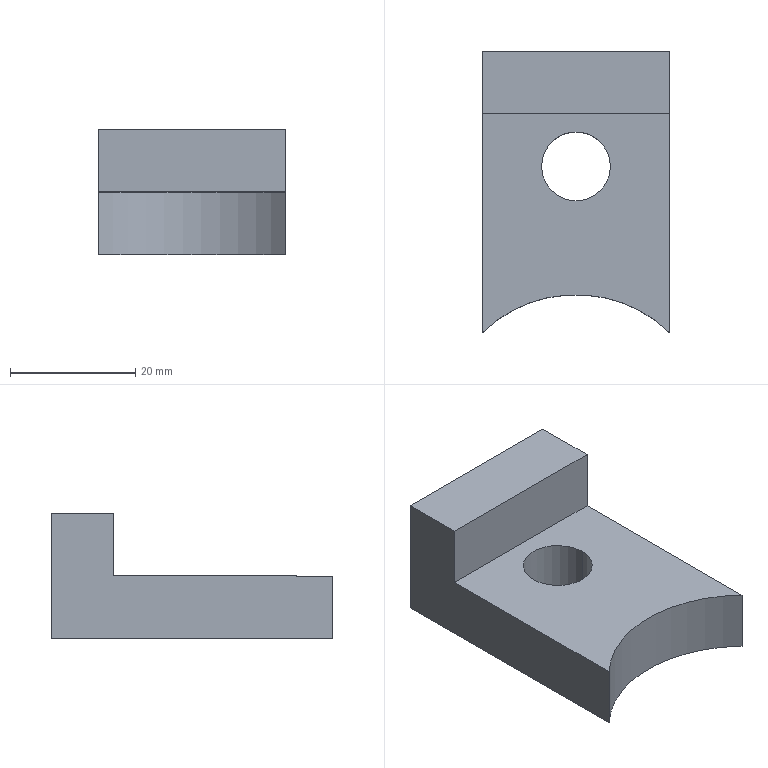Component | SolidWorks | DoubleFilmTransport-1_FlangeClamp-1 | 1 solid | 10 faces | box 30 x 45 x 20 mm | volume 14291 mm3 | plane 7 | cylinder 3 | commonest cylinder face diameters 11 x2 43 x1
build123d program:
from build123d import *

# Parameters (mm, degrees)
BOSS_EXTRUDE1_DEPTH            = 10
SKETCH2_W                      = 30
SKETCH2_H                      = 10
BOSS_EXTRUDE2_DEPTH            = 10
F_11_0_11_DIAMETER_HOLE1_D     = 11
F_11_0_11_DIAMETER_HOLE1_DEPTH = 20


with BuildPart() as part:
    # Sketch1 → Boss-Extrude1 (new body)
    with BuildSketch(Plane(origin=(10, 0, 0), x_dir=(0, 0, -1), z_dir=(1, 0, 0))):
        with BuildLine():
            Line((-15, 0), (-15, -45))
            ThreePointArc((-15, -45), (0, -38.903), (15, -45))
            Line((15, -45), (15, 0))
            Line((15, 0), (-15, 0))
        make_face()
    extrude(amount=-BOSS_EXTRUDE1_DEPTH)

    # Sketch2 → Boss-Extrude2 (add)
    with BuildSketch(Plane(origin=(10, 0, 0), x_dir=(0, 0, -1), z_dir=(1, 0, 0))):
        with Locations((0, -5)):
            Rectangle(SKETCH2_W, SKETCH2_H)
    extrude(amount=BOSS_EXTRUDE2_DEPTH)

    # 11.0 _11_ Diameter Hole1
    with Locations(Plane.ZY):
        with Locations((0, -18.403)):
            Hole(F_11_0_11_DIAMETER_HOLE1_D / 2, depth=F_11_0_11_DIAMETER_HOLE1_DEPTH)


solid = part.part

# Placed as in the assembly
solid = solid.moved(Location((-384.677, 143.776, 56), (0, -90, 0)))
STEP:
#1=COLOUR_RGB('',0.7922,0.8196,0.9333);
#2=FILL_AREA_STYLE_COLOUR('',#1);
#3=FILL_AREA_STYLE('',(#2));
#4=SURFACE_STYLE_FILL_AREA(#3);
#5=SURFACE_SIDE_STYLE('',(#4));
#6=SURFACE_STYLE_USAGE(.BOTH.,#5);
#7=PRESENTATION_STYLE_ASSIGNMENT((#6));
#8=CARTESIAN_POINT('',(-14.928,4.936,2.598));
#9=VERTEX_POINT('',#8);
#10=CARTESIAN_POINT('',(-15.361,4.936,2.598));
#11=VERTEX_POINT('',#10);
#12=CARTESIAN_POINT('',(-15.145,4.936,2.598));
#13=DIRECTION('',(-0.,0.,-1.));
#14=DIRECTION('',(-1.,0.,0.));
#15=AXIS2_PLACEMENT_3D('',#12,#13,#14);
#16=CIRCLE('',#15,0.2165);
#17=EDGE_CURVE('',#9,#11,#16,.T.);
#18=ORIENTED_EDGE('',*,*,#17,.F.);
#19=CARTESIAN_POINT('',(-14.928,4.936,2.205));
#20=VERTEX_POINT('',#19);
#21=CARTESIAN_POINT('',(-14.928,4.936,2.205));
#22=DIRECTION('',(-0.,0.,-1.));
#23=VECTOR('',#22,39.37);
#24=LINE('',#21,#23);
#25=EDGE_CURVE('',#9,#20,#24,.T.);
#26=ORIENTED_EDGE('',*,*,#25,.T.);
#27=CARTESIAN_POINT('',(-15.361,4.936,2.205));
#28=VERTEX_POINT('',#27);
#29=CARTESIAN_POINT('',(-15.145,4.936,2.205));
#30=DIRECTION('',(-0.,0.,-1.));
#31=DIRECTION('',(-1.,0.,0.));
#32=AXIS2_PLACEMENT_3D('',#29,#30,#31);
#33=CIRCLE('',#32,0.2165);
#34=EDGE_CURVE('',#20,#28,#33,.T.);
#35=ORIENTED_EDGE('',*,*,#34,.T.);
#36=CARTESIAN_POINT('',(-15.361,4.936,2.205));
#37=DIRECTION('',(-0.,0.,-1.));
#38=VECTOR('',#37,39.37);
#39=LINE('',#36,#38);
#40=EDGE_CURVE('',#11,#28,#39,.T.);
#41=ORIENTED_EDGE('',*,*,#40,.F.);
#42=EDGE_LOOP('',(#18,#26,#35,#41));
#43=FACE_OUTER_BOUND('',#42,.T.);
#44=CARTESIAN_POINT('',(-15.145,4.936,2.205));
#45=DIRECTION('',(-0.,0.,-1.));
#46=DIRECTION('',(-1.,0.,0.));
#47=AXIS2_PLACEMENT_3D('',#44,#45,#46);
#48=CYLINDRICAL_SURFACE('',#47,0.2165);
#49=ADVANCED_FACE('',(#43),#48,.F.);
#50=CARTESIAN_POINT('',(-15.145,4.936,2.598));
#51=DIRECTION('',(-0.,0.,-1.));
#52=DIRECTION('',(-1.,0.,0.));
#53=AXIS2_PLACEMENT_3D('',#50,#51,#52);
#54=CIRCLE('',#53,0.2165);
#55=EDGE_CURVE('',#11,#9,#54,.T.);
#56=ORIENTED_EDGE('',*,*,#55,.T.);
#57=ORIENTED_EDGE('',*,*,#17,.T.);
#58=EDGE_LOOP('',(#56,#57));
#59=FACE_BOUND('',#58,.T.);
#60=CARTESIAN_POINT('',(-15.735,5.267,2.598));
#61=VERTEX_POINT('',#60);
#62=CARTESIAN_POINT('',(-14.554,5.267,2.598));
#63=VERTEX_POINT('',#62);
#64=CARTESIAN_POINT('',(-14.554,5.267,2.598));
#65=DIRECTION('',(1.,0.,0.));
#66=VECTOR('',#65,39.37);
#67=LINE('',#64,#66);
#68=EDGE_CURVE('',#61,#63,#67,.T.);
#69=ORIENTED_EDGE('',*,*,#68,.F.);
#70=CARTESIAN_POINT('',(-15.735,3.889,2.598));
#71=VERTEX_POINT('',#70);
#72=CARTESIAN_POINT('',(-15.735,5.66,2.598));
#73=DIRECTION('',(0.,-1.,-0.));
#74=VECTOR('',#73,39.37);
#75=LINE('',#72,#74);
#76=EDGE_CURVE('',#61,#71,#75,.T.);
#77=ORIENTED_EDGE('',*,*,#76,.T.);
#78=CARTESIAN_POINT('',(-14.554,3.889,2.598));
#79=VERTEX_POINT('',#78);
#80=CARTESIAN_POINT('',(-15.145,3.282,2.598));
#81=DIRECTION('',(-0.,0.,-1.));
#82=DIRECTION('',(-1.,0.,0.));
#83=AXIS2_PLACEMENT_3D('',#80,#81,#82);
#84=CIRCLE('',#83,0.8465);
#85=EDGE_CURVE('',#71,#79,#84,.T.);
#86=ORIENTED_EDGE('',*,*,#85,.T.);
#87=CARTESIAN_POINT('',(-14.554,3.889,2.598));
#88=DIRECTION('',(-0.,1.,0.));
#89=VECTOR('',#88,39.37);
#90=LINE('',#87,#89);
#91=EDGE_CURVE('',#79,#63,#90,.T.);
#92=ORIENTED_EDGE('',*,*,#91,.T.);
#93=EDGE_LOOP('',(#69,#77,#86,#92));
#94=FACE_OUTER_BOUND('',#93,.T.);
#95=CARTESIAN_POINT('',(-15.145,3.282,2.598));
#96=DIRECTION('',(-0.,0.,-1.));
#97=DIRECTION('',(-1.,-0.,0.));
#98=AXIS2_PLACEMENT_3D('',#95,#96,#97);
#99=PLANE('',#98);
#100=ADVANCED_FACE('',(#59,#94),#99,.F.);
#101=CARTESIAN_POINT('',(-15.735,5.66,2.205));
#102=VERTEX_POINT('',#101);
#103=CARTESIAN_POINT('',(-15.735,5.66,2.992));
#104=VERTEX_POINT('',#103);
#105=CARTESIAN_POINT('',(-15.735,5.66,2.205));
#106=DIRECTION('',(0.,-0.,1.));
#107=VECTOR('',#106,39.37);
#108=LINE('',#105,#107);
#109=EDGE_CURVE('',#102,#104,#108,.T.);
#110=ORIENTED_EDGE('',*,*,#109,.T.);
#111=CARTESIAN_POINT('',(-14.554,5.66,2.992));
#112=VERTEX_POINT('',#111);
#113=CARTESIAN_POINT('',(-15.735,5.66,2.992));
#114=DIRECTION('',(-1.,-0.,0.));
#115=VECTOR('',#114,39.37);
#116=LINE('',#113,#115);
#117=EDGE_CURVE('',#112,#104,#116,.T.);
#118=ORIENTED_EDGE('',*,*,#117,.F.);
#119=CARTESIAN_POINT('',(-14.554,5.66,2.205));
#120=VERTEX_POINT('',#119);
#121=CARTESIAN_POINT('',(-14.554,5.66,2.205));
#122=DIRECTION('',(0.,-0.,1.));
#123=VECTOR('',#122,39.37);
#124=LINE('',#121,#123);
#125=EDGE_CURVE('',#120,#112,#124,.T.);
#126=ORIENTED_EDGE('',*,*,#125,.F.);
#127=CARTESIAN_POINT('',(-14.554,5.66,2.205));
#128=DIRECTION('',(-1.,-0.,0.));
#129=VECTOR('',#128,39.37);
#130=LINE('',#127,#129);
#131=EDGE_CURVE('',#120,#102,#130,.T.);
#132=ORIENTED_EDGE('',*,*,#131,.T.);
#133=EDGE_LOOP('',(#110,#118,#126,#132));
#134=FACE_OUTER_BOUND('',#133,.T.);
#135=CARTESIAN_POINT('',(-14.554,5.66,2.205));
#136=DIRECTION('',(-0.,1.,0.));
#137=DIRECTION('',(-1.,-0.,0.));
#138=AXIS2_PLACEMENT_3D('',#135,#136,#137);
#139=PLANE('',#138);
#140=ADVANCED_FACE('',(#134),#139,.T.);
#141=ORIENTED_EDGE('',*,*,#91,.F.);
#142=CARTESIAN_POINT('',(-14.554,3.889,2.205));
#143=VERTEX_POINT('',#142);
#144=CARTESIAN_POINT('',(-14.554,3.889,2.205));
#145=DIRECTION('',(0.,-0.,1.));
#146=VECTOR('',#145,39.37);
#147=LINE('',#144,#146);
#148=EDGE_CURVE('',#143,#79,#147,.T.);
#149=ORIENTED_EDGE('',*,*,#148,.F.);
#150=CARTESIAN_POINT('',(-14.554,3.889,2.205));
#151=DIRECTION('',(-0.,1.,0.));
#152=VECTOR('',#151,39.37);
#153=LINE('',#150,#152);
#154=EDGE_CURVE('',#143,#120,#153,.T.);
#155=ORIENTED_EDGE('',*,*,#154,.T.);
#156=ORIENTED_EDGE('',*,*,#125,.T.);
#157=CARTESIAN_POINT('',(-14.554,5.267,2.992));
#158=VERTEX_POINT('',#157);
#159=CARTESIAN_POINT('',(-14.554,5.66,2.992));
#160=DIRECTION('',(-0.,1.,0.));
#161=VECTOR('',#160,39.37);
#162=LINE('',#159,#161);
#163=EDGE_CURVE('',#158,#112,#162,.T.);
#164=ORIENTED_EDGE('',*,*,#163,.F.);
#165=CARTESIAN_POINT('',(-14.554,5.267,2.992));
#166=DIRECTION('',(-0.,0.,-1.));
#167=VECTOR('',#166,39.37);
#168=LINE('',#165,#167);
#169=EDGE_CURVE('',#158,#63,#168,.T.);
#170=ORIENTED_EDGE('',*,*,#169,.T.);
#171=EDGE_LOOP('',(#141,#149,#155,#156,#164,#170));
#172=FACE_OUTER_BOUND('',#171,.T.);
#173=CARTESIAN_POINT('',(-14.554,3.889,2.205));
#174=DIRECTION('',(1.,0.,-0.));
#175=DIRECTION('',(-0.,0.,-1.));
#176=AXIS2_PLACEMENT_3D('',#173,#174,#175);
#177=PLANE('',#176);
#178=ADVANCED_FACE('',(#172),#177,.T.);
#179=ORIENTED_EDGE('',*,*,#85,.F.);
#180=CARTESIAN_POINT('',(-15.735,3.889,2.205));
#181=VERTEX_POINT('',#180);
#182=CARTESIAN_POINT('',(-15.735,3.889,2.205));
#183=DIRECTION('',(0.,-0.,1.));
#184=VECTOR('',#183,39.37);
#185=LINE('',#182,#184);
#186=EDGE_CURVE('',#181,#71,#185,.T.);
#187=ORIENTED_EDGE('',*,*,#186,.F.);
#188=CARTESIAN_POINT('',(-15.145,3.282,2.205));
#189=DIRECTION('',(-0.,0.,-1.));
#190=DIRECTION('',(-1.,0.,0.));
#191=AXIS2_PLACEMENT_3D('',#188,#189,#190);
#192=CIRCLE('',#191,0.8465);
#193=EDGE_CURVE('',#181,#143,#192,.T.);
#194=ORIENTED_EDGE('',*,*,#193,.T.);
#195=ORIENTED_EDGE('',*,*,#148,.T.);
#196=EDGE_LOOP('',(#179,#187,#194,#195));
#197=FACE_OUTER_BOUND('',#196,.T.);
#198=CARTESIAN_POINT('',(-15.145,3.282,2.205));
#199=DIRECTION('',(0.,-0.,1.));
#200=DIRECTION('',(1.,0.,0.));
#201=AXIS2_PLACEMENT_3D('',#198,#199,#200);
#202=CYLINDRICAL_SURFACE('',#201,0.8465);
#203=ADVANCED_FACE('',(#197),#202,.F.);
#204=ORIENTED_EDGE('',*,*,#76,.F.);
#205=CARTESIAN_POINT('',(-15.735,5.267,2.992));
#206=VERTEX_POINT('',#205);
#207=CARTESIAN_POINT('',(-15.735,5.267,2.992));
#208=DIRECTION('',(-0.,0.,-1.));
#209=VECTOR('',#208,39.37);
#210=LINE('',#207,#209);
#211=EDGE_CURVE('',#206,#61,#210,.T.);
#212=ORIENTED_EDGE('',*,*,#211,.F.);
#213=CARTESIAN_POINT('',(-15.735,5.267,2.992));
#214=DIRECTION('',(0.,-1.,-0.));
#215=VECTOR('',#214,39.37);
#216=LINE('',#213,#215);
#217=EDGE_CURVE('',#104,#206,#216,.T.);
#218=ORIENTED_EDGE('',*,*,#217,.F.);
#219=ORIENTED_EDGE('',*,*,#109,.F.);
#220=CARTESIAN_POINT('',(-15.735,5.66,2.205));
#221=DIRECTION('',(0.,-1.,-0.));
#222=VECTOR('',#221,39.37);
#223=LINE('',#220,#222);
#224=EDGE_CURVE('',#102,#181,#223,.T.);
#225=ORIENTED_EDGE('',*,*,#224,.T.);
#226=ORIENTED_EDGE('',*,*,#186,.T.);
#227=EDGE_LOOP('',(#204,#212,#218,#219,#225,#226));
#228=FACE_OUTER_BOUND('',#227,.T.);
#229=CARTESIAN_POINT('',(-15.735,5.66,2.205));
#230=DIRECTION('',(-1.,-0.,-0.));
#231=DIRECTION('',(0.,-1.,-0.));
#232=AXIS2_PLACEMENT_3D('',#229,#230,#231);
#233=PLANE('',#232);
#234=ADVANCED_FACE('',(#228),#233,.T.);
#235=CARTESIAN_POINT('',(-15.145,4.936,2.205));
#236=DIRECTION('',(-0.,0.,-1.));
#237=DIRECTION('',(-1.,0.,0.));
#238=AXIS2_PLACEMENT_3D('',#235,#236,#237);
#239=CIRCLE('',#238,0.2165);
#240=EDGE_CURVE('',#28,#20,#239,.T.);
#241=ORIENTED_EDGE('',*,*,#240,.F.);
#242=ORIENTED_EDGE('',*,*,#34,.F.);
#243=EDGE_LOOP('',(#241,#242));
#244=FACE_BOUND('',#243,.T.);
#245=ORIENTED_EDGE('',*,*,#131,.F.);
#246=ORIENTED_EDGE('',*,*,#154,.F.);
#247=ORIENTED_EDGE('',*,*,#193,.F.);
#248=ORIENTED_EDGE('',*,*,#224,.F.);
#249=EDGE_LOOP('',(#245,#246,#247,#248));
#250=FACE_OUTER_BOUND('',#249,.T.);
#251=CARTESIAN_POINT('',(-15.145,3.282,2.205));
#252=DIRECTION('',(-0.,0.,-1.));
#253=DIRECTION('',(-1.,-0.,0.));
#254=AXIS2_PLACEMENT_3D('',#251,#252,#253);
#255=PLANE('',#254);
#256=ADVANCED_FACE('',(#244,#250),#255,.T.);
#257=ORIENTED_EDGE('',*,*,#68,.T.);
#258=ORIENTED_EDGE('',*,*,#169,.F.);
#259=CARTESIAN_POINT('',(-14.554,5.267,2.992));
#260=DIRECTION('',(1.,0.,0.));
#261=VECTOR('',#260,39.37);
#262=LINE('',#259,#261);
#263=EDGE_CURVE('',#206,#158,#262,.T.);
#264=ORIENTED_EDGE('',*,*,#263,.F.);
#265=ORIENTED_EDGE('',*,*,#211,.T.);
#266=EDGE_LOOP('',(#257,#258,#264,#265));
#267=FACE_OUTER_BOUND('',#266,.T.);
#268=CARTESIAN_POINT('',(-14.554,5.267,2.992));
#269=DIRECTION('',(-0.,1.,0.));
#270=DIRECTION('',(-1.,-0.,0.));
#271=AXIS2_PLACEMENT_3D('',#268,#269,#270);
#272=PLANE('',#271);
#273=ADVANCED_FACE('',(#267),#272,.F.);
#274=ORIENTED_EDGE('',*,*,#263,.T.);
#275=ORIENTED_EDGE('',*,*,#163,.T.);
#276=ORIENTED_EDGE('',*,*,#117,.T.);
#277=ORIENTED_EDGE('',*,*,#217,.T.);
#278=EDGE_LOOP('',(#274,#275,#276,#277));
#279=FACE_OUTER_BOUND('',#278,.T.);
#280=CARTESIAN_POINT('',(-15.145,5.66,2.992));
#281=DIRECTION('',(-0.,0.,-1.));
#282=DIRECTION('',(-1.,-0.,0.));
#283=AXIS2_PLACEMENT_3D('',#280,#281,#282);
#284=PLANE('',#283);
#285=ADVANCED_FACE('',(#279),#284,.F.);
#286=ORIENTED_EDGE('',*,*,#25,.F.);
#287=ORIENTED_EDGE('',*,*,#55,.F.);
#288=ORIENTED_EDGE('',*,*,#40,.T.);
#289=ORIENTED_EDGE('',*,*,#240,.T.);
#290=EDGE_LOOP('',(#286,#287,#288,#289));
#291=FACE_OUTER_BOUND('',#290,.T.);
#292=CARTESIAN_POINT('',(-15.145,4.936,2.205));
#293=DIRECTION('',(-0.,0.,-1.));
#294=DIRECTION('',(-1.,0.,0.));
#295=AXIS2_PLACEMENT_3D('',#292,#293,#294);
#296=CYLINDRICAL_SURFACE('',#295,0.2165);
#297=ADVANCED_FACE('',(#291),#296,.F.);
#298=CLOSED_SHELL('',(#49,#100,#140,#178,#203,#234,#256,#273,#285,#297));
#299=MANIFOLD_SOLID_BREP('',#298);
#300=STYLED_ITEM('',(#7),#299);
#301=(LENGTH_UNIT()NAMED_UNIT(*)SI_UNIT($,.METRE.));
#302=LENGTH_MEASURE_WITH_UNIT(LENGTH_MEASURE(0.0254),#301);
#303=DIMENSIONAL_EXPONENTS(1.,0.,0.,0.,0.,0.,0.);
#304=(CONVERSION_BASED_UNIT('',#302)LENGTH_UNIT()NAMED_UNIT(#303));
#305=UNCERTAINTY_MEASURE_WITH_UNIT(LENGTH_MEASURE(0.00001),#304,'','');
#306=(NAMED_UNIT(*)PLANE_ANGLE_UNIT()SI_UNIT($,.RADIAN.));
#307=(NAMED_UNIT(*)SI_UNIT($,.STERADIAN.)SOLID_ANGLE_UNIT());
#308=(GEOMETRIC_REPRESENTATION_CONTEXT(3)GLOBAL_UNCERTAINTY_ASSIGNED_CONTEXT((#305))GLOBAL_UNIT_ASSIGNED_CONTEXT((#304,#306,#307))REPRESENTATION_CONTEXT('',''));
#309=MECHANICAL_DESIGN_GEOMETRIC_PRESENTATION_REPRESENTATION('',(#300),#308);
#310=CARTESIAN_POINT('',(0.,0.,0.));
#311=DIRECTION('',(0.,0.,1.));
#312=DIRECTION('',(1.,0.,0.));
#313=AXIS2_PLACEMENT_3D('',#310,#311,#312);
#314=(LENGTH_UNIT()NAMED_UNIT(*)SI_UNIT($,.METRE.));
#315=LENGTH_MEASURE_WITH_UNIT(LENGTH_MEASURE(0.0254),#314);
#316=DIMENSIONAL_EXPONENTS(1.,0.,0.,0.,0.,0.,0.);
#317=(CONVERSION_BASED_UNIT('',#315)LENGTH_UNIT()NAMED_UNIT(#316));
#318=UNCERTAINTY_MEASURE_WITH_UNIT(LENGTH_MEASURE(0.00001),#317,'','');
#319=(NAMED_UNIT(*)PLANE_ANGLE_UNIT()SI_UNIT($,.RADIAN.));
#320=(NAMED_UNIT(*)SI_UNIT($,.STERADIAN.)SOLID_ANGLE_UNIT());
#321=(GEOMETRIC_REPRESENTATION_CONTEXT(3)GLOBAL_UNCERTAINTY_ASSIGNED_CONTEXT((#318))GLOBAL_UNIT_ASSIGNED_CONTEXT((#317,#319,#320))REPRESENTATION_CONTEXT('',''));
#322=ADVANCED_BREP_SHAPE_REPRESENTATION('',(#299,#313),#321);
#323=PRESENTATION_LAYER_ASSIGNMENT('','',(#300));